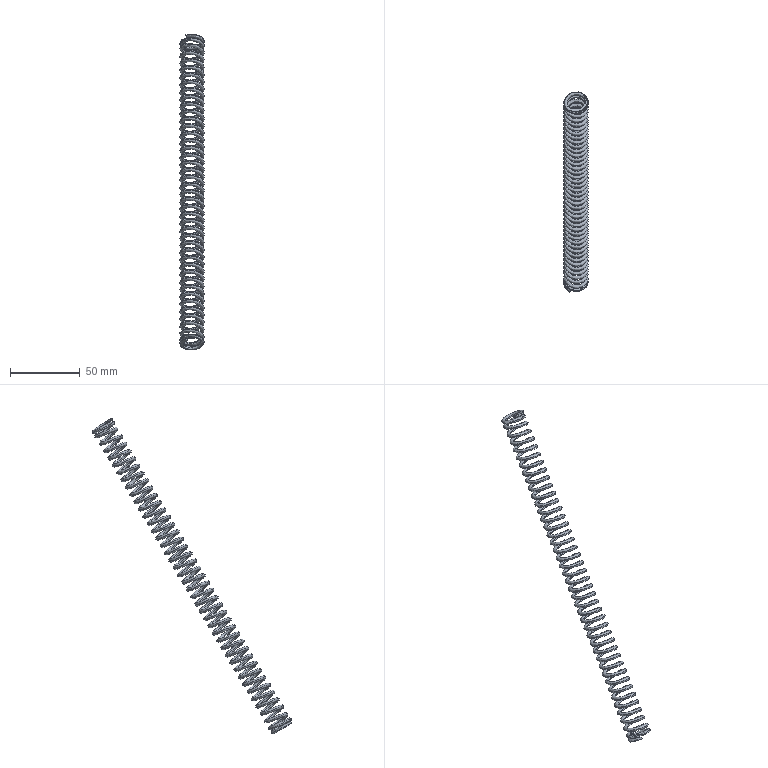Component | SolidWorks | Spring2-1 | 1 solid | 6 faces | volume 10079 mm3 | plane 4 | spline 2